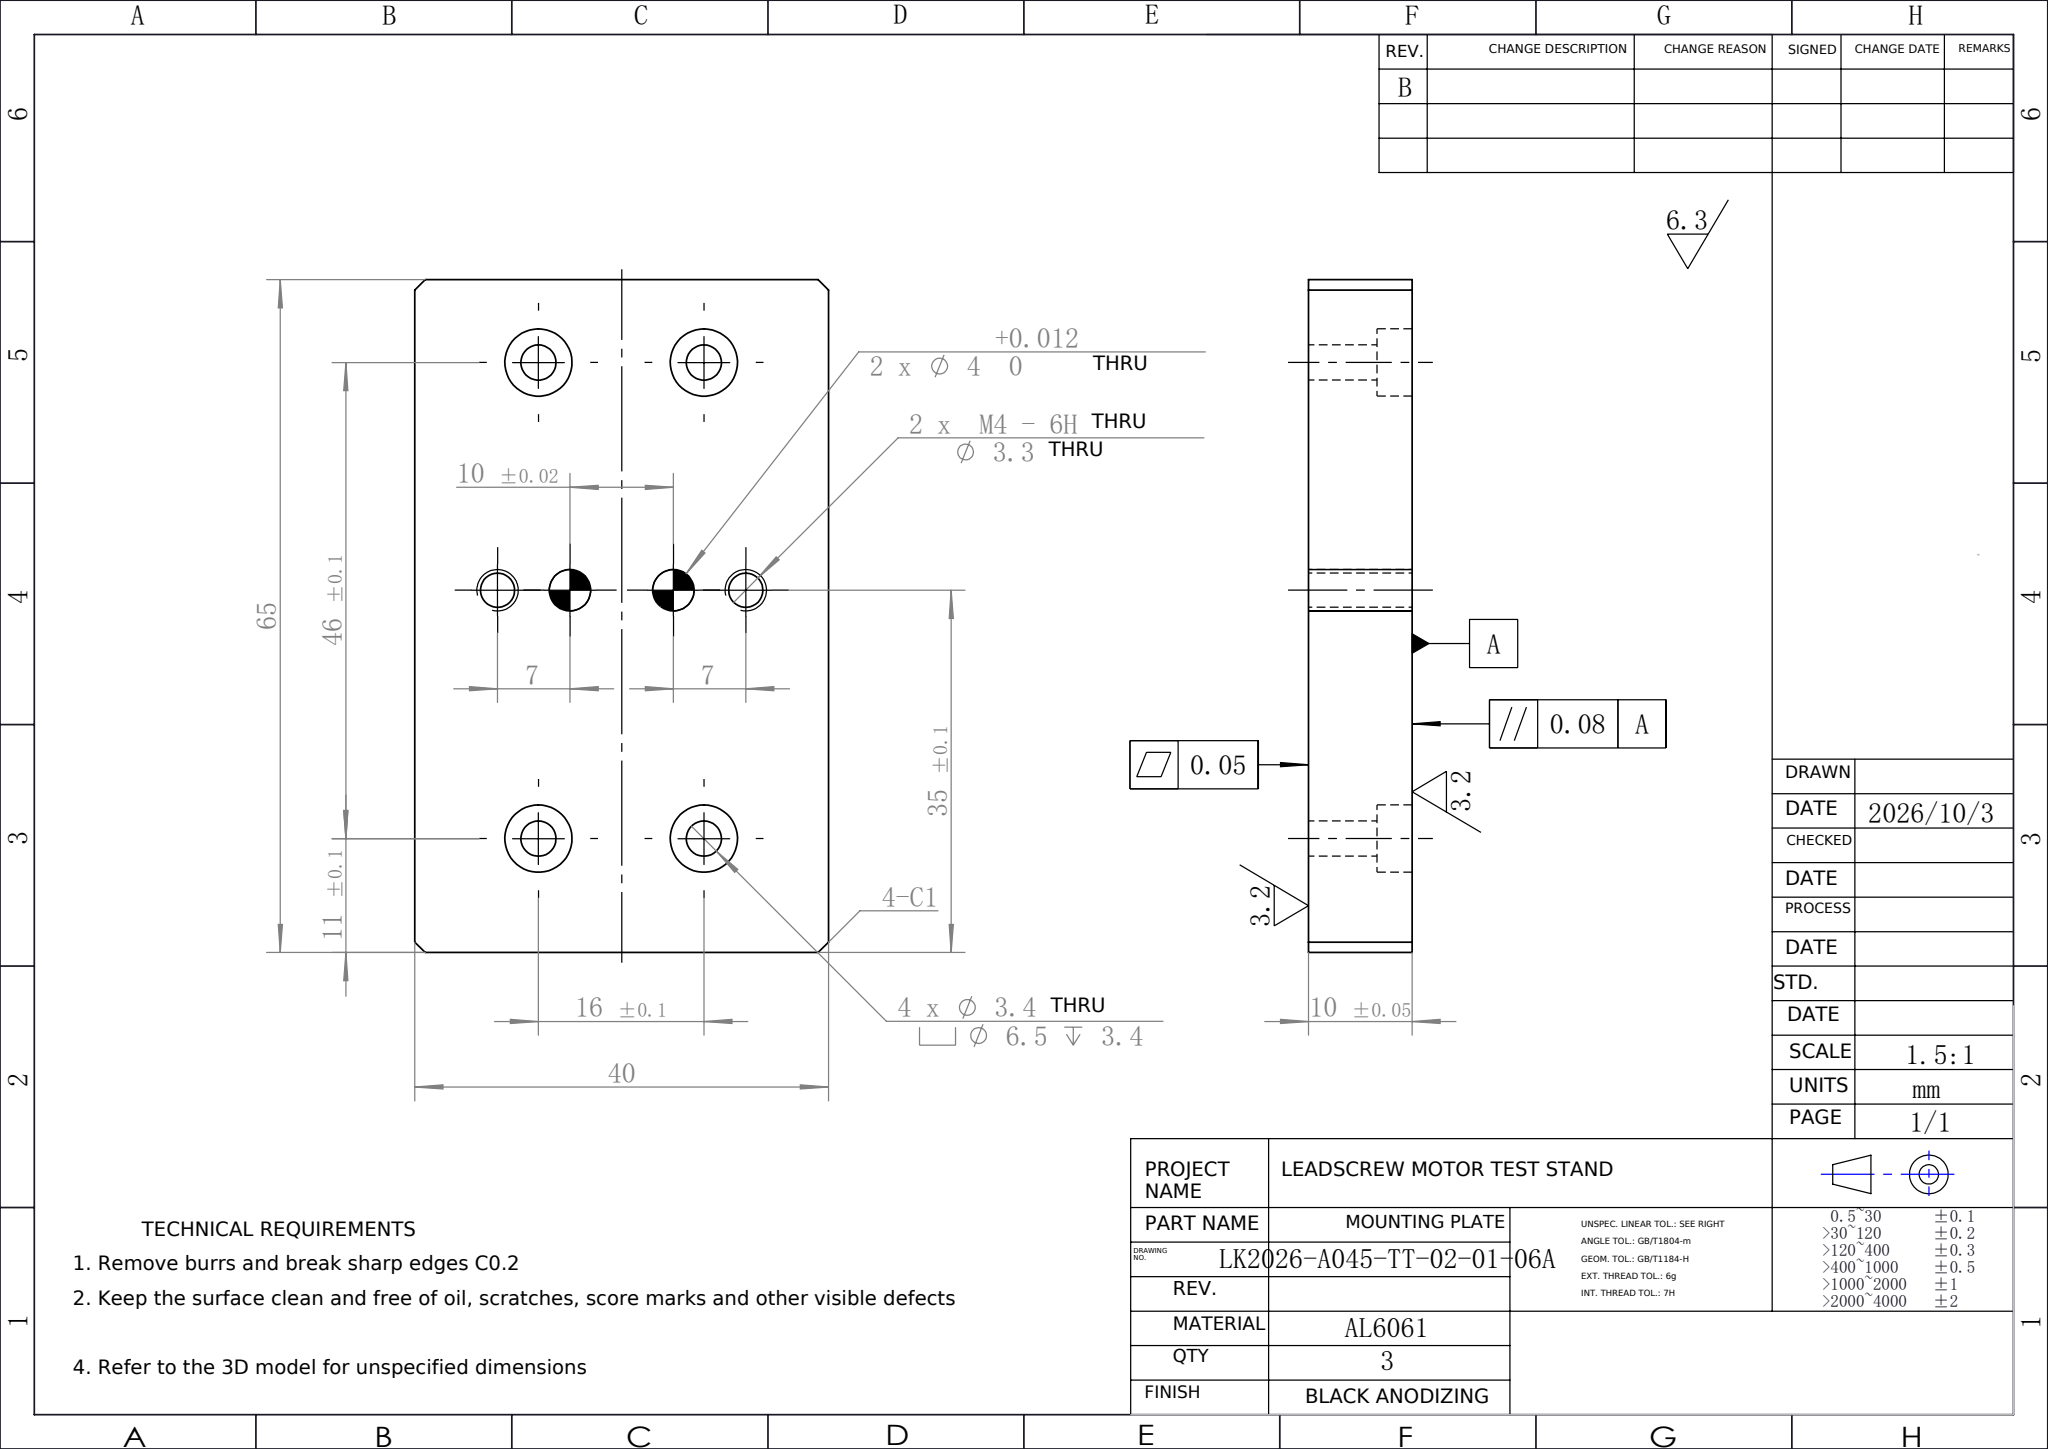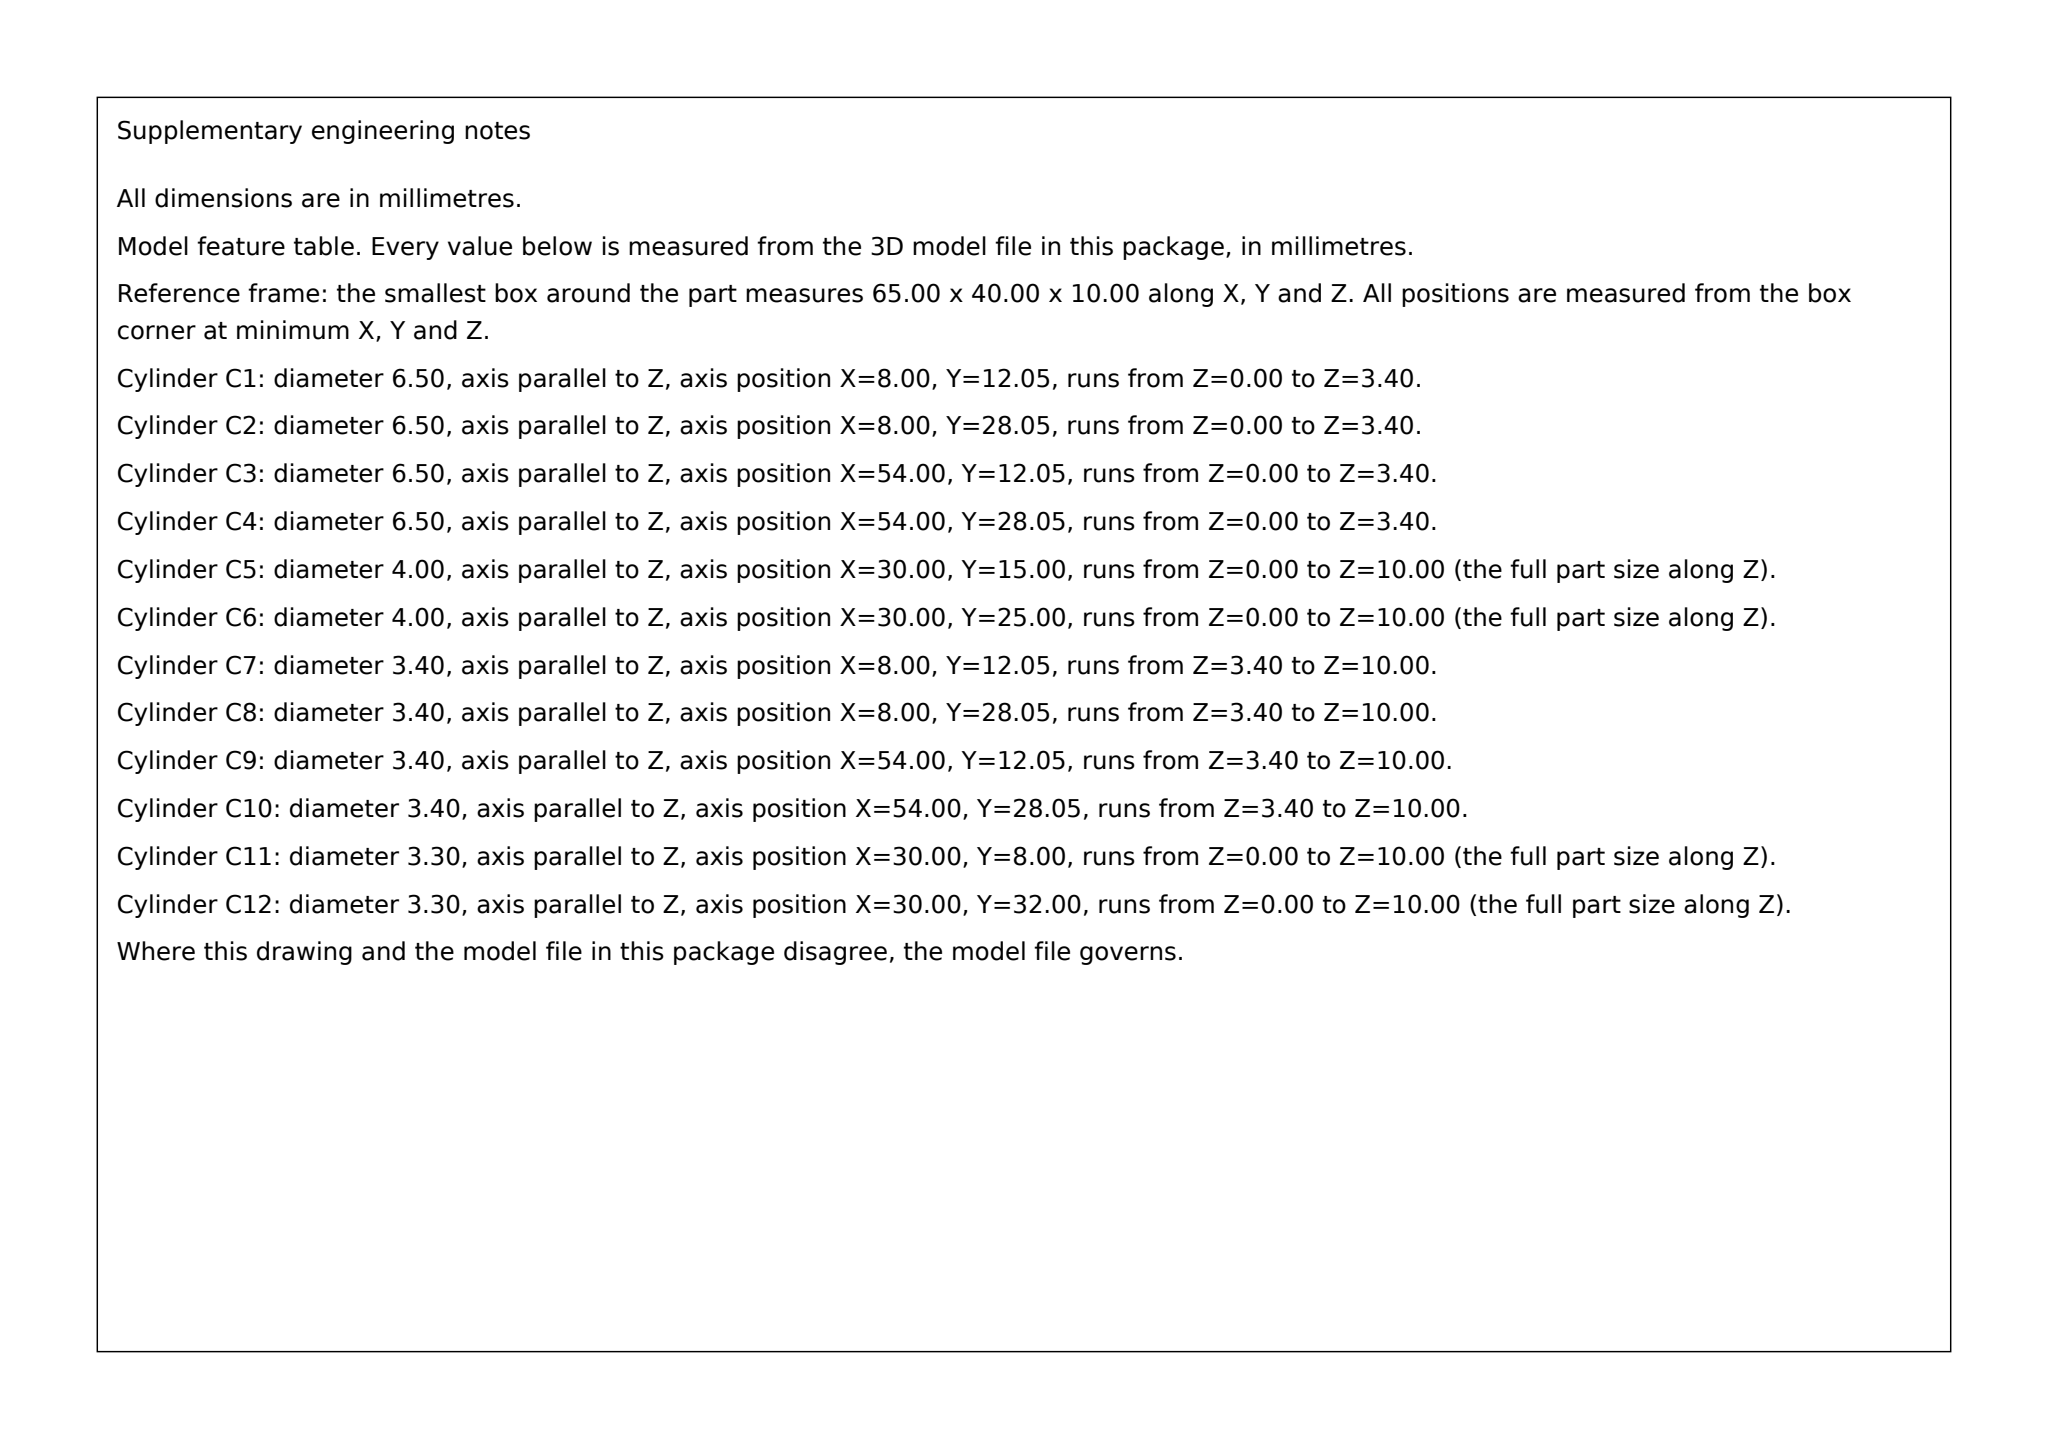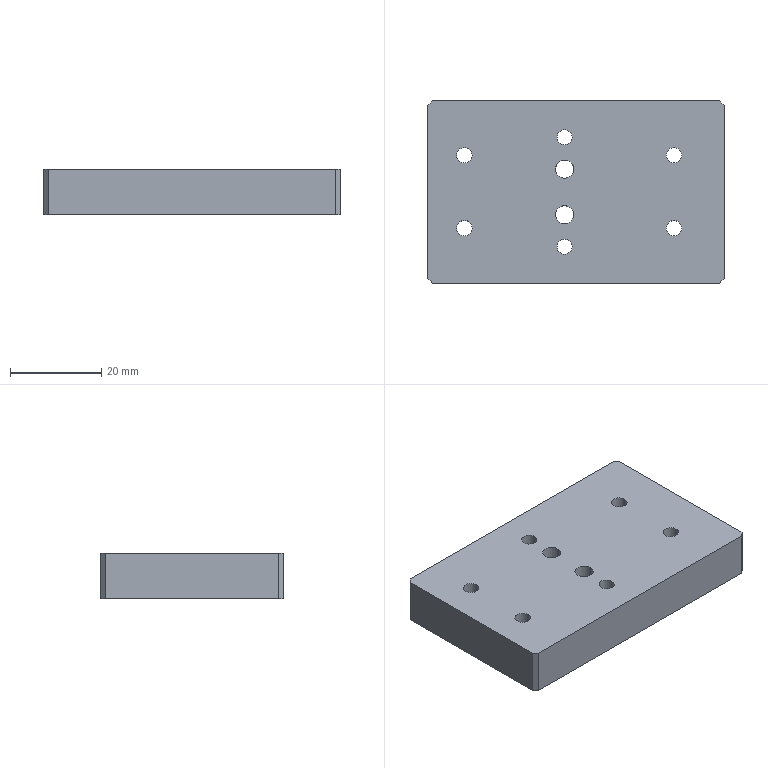Part | SolidWorks | mm | 1 solid | 38 faces | box 65 x 40 x 10 mm | volume 24867 mm3 | cylinder 24 | plane 14 | commonest cylinder face diameters 6.5 x8 3.4 x8 4 x4 3.3 x4
build123d program:
from build123d import *

# Parameters (mm, degrees)
SKETCH1_W                                       = 65
SKETCH1_H                                       = 40
BOSS_EXTRUDE1_DEPTH                             = 5
CHAMFER1_SIZE                                   = 1
M4_TAPPED_HOLE1_D                               = 3.3
F_4_0_MM_DOWEL_PIN_HOLE1_D                      = 4
M3_HEX_SOCKET_HEAD_CAP_SCREW_CBORE1_D           = 3.4
M3_HEX_SOCKET_HEAD_CAP_SCREW_CBORE1_CBORE_D     = 6.5
M3_HEX_SOCKET_HEAD_CAP_SCREW_CBORE1_CBORE_DEPTH = 3.4


with BuildPart() as part:
    # Sketch1 → Boss-Extrude1 (new, symmetric)
    with BuildSketch(Plane.XY):
        Rectangle(SKETCH1_W, SKETCH1_H)
    extrude(amount=BOSS_EXTRUDE1_DEPTH, both=True)

    # Chamfer1
    chamfer1_edges = [part.edges().sort_by_distance(p)[0] for p in [
        (32.5, -20, 0),
        (-32.5, -20, 0),
        (-32.5, 20, 0),
        (32.5, 20, 0),
    ]]
    chamfer(chamfer1_edges, length=CHAMFER1_SIZE)

    # M4 Tapped Hole1 (through all)
    with Locations(Plane(origin=(0, 0, -5), x_dir=(-1, 0, 0), z_dir=(0, 0, -1))):
        with Locations((2.5, 12), (2.5, -12)):
            Hole(M4_TAPPED_HOLE1_D / 2)

    # 4.0 mm Dowel Pin Hole1 (through all)
    with Locations(Plane(origin=(0, 0, -5), x_dir=(-1, 0, 0), z_dir=(0, 0, -1))):
        with Locations((2.5, -5), (2.5, 5)):
            Hole(F_4_0_MM_DOWEL_PIN_HOLE1_D / 2)

    # M3 Hex Socket Head Cap Screw CBORE1 (through all)
    with Locations(Plane(origin=(0, 0, -5), x_dir=(-1, 0, 0), z_dir=(0, 0, -1))):
        with Locations((-21.5, -7.95), (-21.5, 8.05), (24.5, 8.05), (24.5, -7.95)):
            CounterBoreHole(M3_HEX_SOCKET_HEAD_CAP_SCREW_CBORE1_D / 2, M3_HEX_SOCKET_HEAD_CAP_SCREW_CBORE1_CBORE_D / 2, M3_HEX_SOCKET_HEAD_CAP_SCREW_CBORE1_CBORE_DEPTH)


solid = part.part